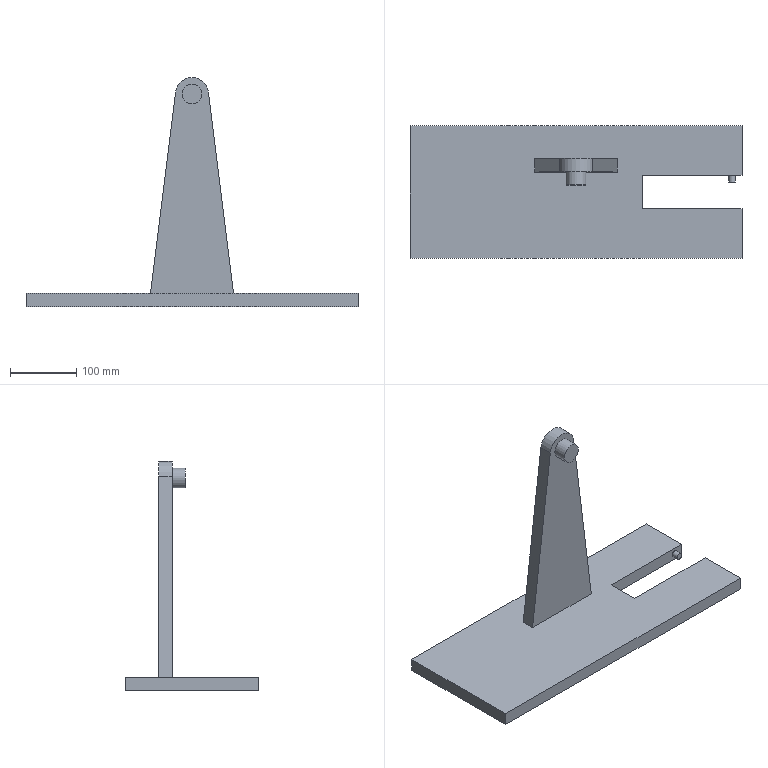Component | NX | STAND | 1 solid | 19 faces | volume 2410721 mm3 | plane 16 | cylinder 3 | commonest cylinder face diameters 50 x1 30 x1 10 x1